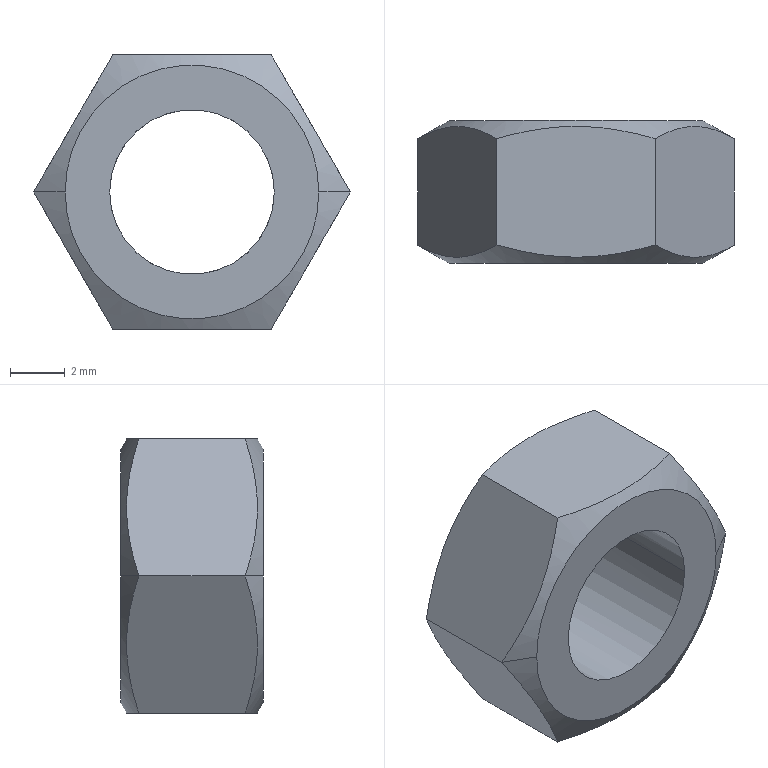Component | SolidWorks | hex nuts, style 1-grades ab gb-1 | 1 solid | 14 faces | volume 295 mm3 | plane 8 | cone 4 | cylinder 2 | commonest cylinder face diameters 6 x2